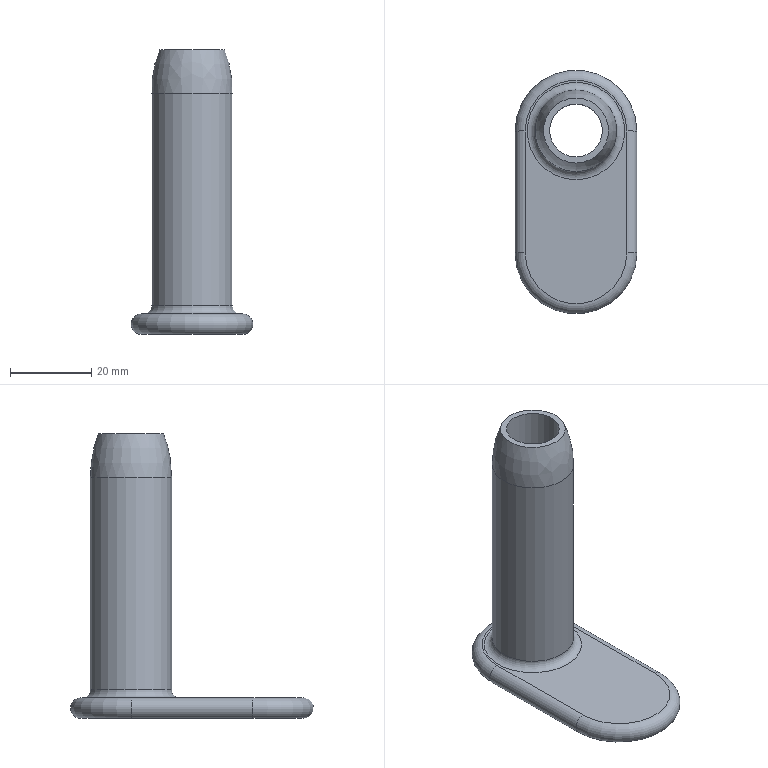Component | NX | UPPER_MOUNT_2 | 1 solid | 14 faces | box 30 x 60 x 70 mm | volume 13408 mm3 | cylinder 5 | plane 3 | torus 3 | cone 2 | spline 1 | commonest cylinder face diameters 5 x2 20 x1 18 x1 13 x1
STEP:
#1=CARTESIAN_POINT('',(0.,0.,0.));
#2=DIRECTION('',(0.,0.,1.));
#3=DIRECTION('',(1.,0.,0.));
#4=AXIS2_PLACEMENT_3D('',#1,#2,#3);
#5=CARTESIAN_POINT('',(-270.,134.875,-190.));
#6=VERTEX_POINT('',#5);
#7=CARTESIAN_POINT('',(-270.,124.875,-190.));
#8=DIRECTION('',(0.,0.,1.));
#9=DIRECTION('',(0.,1.,0.));
#10=AXIS2_PLACEMENT_3D('',#7,#8,#9);
#11=CIRCLE('',#10,10.);
#12=CARTESIAN_POINT('',(-270.,94.875,-190.));
#13=DIRECTION('',(0.,0.,1.));
#14=DIRECTION('',(0.,1.,0.));
#15=AXIS2_PLACEMENT_3D('',#12,#13,#14);
#16=PLANE('',#15);
#17=CARTESIAN_POINT('',(30.,0.));
#18=DIRECTION('',(1.,0.));
#19=AXIS2_PLACEMENT_2D('',#17,#18);
#20=CIRCLE('',#19,10.);
#21=(GEOMETRIC_REPRESENTATION_CONTEXT(2)PARAMETRIC_REPRESENTATION_CONTEXT()REPRESENTATION_CONTEXT('',''));
#22=DEFINITIONAL_REPRESENTATION('',(#20),#21);
#23=PCURVE('',#16,#22);
#24=CARTESIAN_POINT('',(-270.,124.875,-190.));
#25=DIRECTION('',(0.,0.,-1.));
#26=DIRECTION('',(0.,-1.,0.));
#27=AXIS2_PLACEMENT_3D('',#24,#25,#26);
#28=CONICAL_SURFACE('',#27,10.,0.7854);
#29=CARTESIAN_POINT('',(9.425,0.));
#30=DIRECTION('',(-1.,0.));
#31=VECTOR('',#30,1.);
#32=LINE('',#29,#31);
#33=(GEOMETRIC_REPRESENTATION_CONTEXT(2)PARAMETRIC_REPRESENTATION_CONTEXT()REPRESENTATION_CONTEXT('',''));
#34=DEFINITIONAL_REPRESENTATION('',(#32),#33);
#35=PCURVE('',#28,#34);
#36=SURFACE_CURVE('',#11,(#23,#35),.PCURVE_S1.);
#37=EDGE_CURVE('',#6,#6,#36,.T.);
#38=ORIENTED_EDGE('',*,*,#37,.T.);
#39=EDGE_LOOP('',(#38));
#40=FACE_BOUND('',#39,.T.);
#41=CARTESIAN_POINT('',(-282.5,94.875,-190.));
#42=VERTEX_POINT('',#41);
#43=CARTESIAN_POINT('',(-282.5,124.875,-190.));
#44=VERTEX_POINT('',#43);
#45=CARTESIAN_POINT('',(-282.5,124.875,-190.));
#46=DIRECTION('',(0.,1.,0.));
#47=VECTOR('',#46,1.);
#48=LINE('',#45,#47);
#49=CARTESIAN_POINT('',(30.,12.5));
#50=DIRECTION('',(1.,0.));
#51=VECTOR('',#50,1.);
#52=LINE('',#49,#51);
#53=(GEOMETRIC_REPRESENTATION_CONTEXT(2)PARAMETRIC_REPRESENTATION_CONTEXT()REPRESENTATION_CONTEXT('',''));
#54=DEFINITIONAL_REPRESENTATION('',(#52),#53);
#55=PCURVE('',#16,#54);
#56=CARTESIAN_POINT('',(-282.5,124.875,-187.5));
#57=DIRECTION('',(0.,1.,0.));
#58=DIRECTION('',(0.,0.,-1.));
#59=AXIS2_PLACEMENT_3D('',#56,#57,#58);
#60=CYLINDRICAL_SURFACE('',#59,2.5);
#61=CARTESIAN_POINT('',(0.,0.));
#62=DIRECTION('',(0.,1.));
#63=VECTOR('',#62,1.);
#64=LINE('',#61,#63);
#65=(GEOMETRIC_REPRESENTATION_CONTEXT(2)PARAMETRIC_REPRESENTATION_CONTEXT()REPRESENTATION_CONTEXT('',''));
#66=DEFINITIONAL_REPRESENTATION('',(#64),#65);
#67=PCURVE('',#60,#66);
#68=SURFACE_CURVE('',#48,(#55,#67),.PCURVE_S1.);
#69=EDGE_CURVE('',#42,#44,#68,.T.);
#70=ORIENTED_EDGE('',*,*,#69,.T.);
#71=CARTESIAN_POINT('',(-257.5,124.875,-190.));
#72=VERTEX_POINT('',#71);
#73=CARTESIAN_POINT('',(-270.,124.875,-190.));
#74=DIRECTION('',(0.,0.,-1.));
#75=DIRECTION('',(0.,1.,0.));
#76=AXIS2_PLACEMENT_3D('',#73,#74,#75);
#77=CIRCLE('',#76,12.5);
#78=CARTESIAN_POINT('',(42.5,0.));
#79=CARTESIAN_POINT('',(42.5,-21.651));
#80=CARTESIAN_POINT('',(23.75,-10.825));
#81=CARTESIAN_POINT('',(5.,-0.));
#82=CARTESIAN_POINT('',(23.75,10.825));
#83=CARTESIAN_POINT('',(42.5,21.651));
#84=CARTESIAN_POINT('',(42.5,0.));
#85=(BOUNDED_CURVE()B_SPLINE_CURVE(2,(#78,#79,#80,#81,#82,#83,#84),.UNSPECIFIED.,.T.,.F.)B_SPLINE_CURVE_WITH_KNOTS((1,2,2,2,2,1),(-2.094,0.,2.094,4.189,6.283,8.378),.UNSPECIFIED.)CURVE()GEOMETRIC_REPRESENTATION_ITEM()RATIONAL_B_SPLINE_CURVE((1.,0.5,1.,0.5,1.,0.5,1.))REPRESENTATION_ITEM(''));
#86=(GEOMETRIC_REPRESENTATION_CONTEXT(2)PARAMETRIC_REPRESENTATION_CONTEXT()REPRESENTATION_CONTEXT('',''));
#87=DEFINITIONAL_REPRESENTATION('',(#85),#86);
#88=PCURVE('',#16,#87);
#89=CARTESIAN_POINT('',(-270.,124.875,-187.5));
#90=DIRECTION('',(0.,0.,1.));
#91=DIRECTION('',(0.,1.,0.));
#92=AXIS2_PLACEMENT_3D('',#89,#90,#91);
#93=TOROIDAL_SURFACE('',#92,12.5,2.5);
#94=CARTESIAN_POINT('',(12.566,-1.571));
#95=DIRECTION('',(-1.,0.));
#96=VECTOR('',#95,1.);
#97=LINE('',#94,#96);
#98=(GEOMETRIC_REPRESENTATION_CONTEXT(2)PARAMETRIC_REPRESENTATION_CONTEXT()REPRESENTATION_CONTEXT('',''));
#99=DEFINITIONAL_REPRESENTATION('',(#97),#98);
#100=PCURVE('',#93,#99);
#101=SURFACE_CURVE('',#77,(#88,#100),.PCURVE_S1.);
#102=EDGE_CURVE('',#44,#72,#101,.T.);
#103=ORIENTED_EDGE('',*,*,#102,.T.);
#104=CARTESIAN_POINT('',(-257.5,94.875,-190.));
#105=VERTEX_POINT('',#104);
#106=CARTESIAN_POINT('',(-257.5,94.875,-190.));
#107=DIRECTION('',(0.,-1.,0.));
#108=VECTOR('',#107,1.);
#109=LINE('',#106,#108);
#110=CARTESIAN_POINT('',(0.,-12.5));
#111=DIRECTION('',(-1.,0.));
#112=VECTOR('',#111,1.);
#113=LINE('',#110,#112);
#114=(GEOMETRIC_REPRESENTATION_CONTEXT(2)PARAMETRIC_REPRESENTATION_CONTEXT()REPRESENTATION_CONTEXT('',''));
#115=DEFINITIONAL_REPRESENTATION('',(#113),#114);
#116=PCURVE('',#16,#115);
#117=CARTESIAN_POINT('',(-257.5,94.875,-187.5));
#118=DIRECTION('',(0.,-1.,0.));
#119=DIRECTION('',(0.,0.,1.));
#120=AXIS2_PLACEMENT_3D('',#117,#118,#119);
#121=CYLINDRICAL_SURFACE('',#120,2.5);
#122=CARTESIAN_POINT('',(3.142,0.));
#123=DIRECTION('',(0.,1.));
#124=VECTOR('',#123,1.);
#125=LINE('',#122,#124);
#126=(GEOMETRIC_REPRESENTATION_CONTEXT(2)PARAMETRIC_REPRESENTATION_CONTEXT()REPRESENTATION_CONTEXT('',''));
#127=DEFINITIONAL_REPRESENTATION('',(#125),#126);
#128=PCURVE('',#121,#127);
#129=SURFACE_CURVE('',#109,(#116,#128),.PCURVE_S1.);
#130=EDGE_CURVE('',#72,#105,#129,.T.);
#131=ORIENTED_EDGE('',*,*,#130,.T.);
#132=CARTESIAN_POINT('',(-270.,94.875,-190.));
#133=DIRECTION('',(0.,0.,-1.));
#134=DIRECTION('',(0.,1.,0.));
#135=AXIS2_PLACEMENT_3D('',#132,#133,#134);
#136=CIRCLE('',#135,12.5);
#137=CARTESIAN_POINT('',(12.5,0.));
#138=CARTESIAN_POINT('',(12.5,-21.651));
#139=CARTESIAN_POINT('',(-6.25,-10.825));
#140=CARTESIAN_POINT('',(-25.,-0.));
#141=CARTESIAN_POINT('',(-6.25,10.825));
#142=CARTESIAN_POINT('',(12.5,21.651));
#143=CARTESIAN_POINT('',(12.5,0.));
#144=(BOUNDED_CURVE()B_SPLINE_CURVE(2,(#137,#138,#139,#140,#141,#142,#143),.UNSPECIFIED.,.T.,.F.)B_SPLINE_CURVE_WITH_KNOTS((1,2,2,2,2,1),(-2.094,0.,2.094,4.189,6.283,8.378),.UNSPECIFIED.)CURVE()GEOMETRIC_REPRESENTATION_ITEM()RATIONAL_B_SPLINE_CURVE((1.,0.5,1.,0.5,1.,0.5,1.))REPRESENTATION_ITEM(''));
#145=(GEOMETRIC_REPRESENTATION_CONTEXT(2)PARAMETRIC_REPRESENTATION_CONTEXT()REPRESENTATION_CONTEXT('',''));
#146=DEFINITIONAL_REPRESENTATION('',(#144),#145);
#147=PCURVE('',#16,#146);
#148=CARTESIAN_POINT('',(-270.,94.875,-187.5));
#149=DIRECTION('',(0.,0.,1.));
#150=DIRECTION('',(0.,1.,0.));
#151=AXIS2_PLACEMENT_3D('',#148,#149,#150);
#152=TOROIDAL_SURFACE('',#151,12.5,2.5);
#153=CARTESIAN_POINT('',(6.283,-1.571));
#154=DIRECTION('',(-1.,0.));
#155=VECTOR('',#154,1.);
#156=LINE('',#153,#155);
#157=(GEOMETRIC_REPRESENTATION_CONTEXT(2)PARAMETRIC_REPRESENTATION_CONTEXT()REPRESENTATION_CONTEXT('',''));
#158=DEFINITIONAL_REPRESENTATION('',(#156),#157);
#159=PCURVE('',#152,#158);
#160=SURFACE_CURVE('',#136,(#147,#159),.PCURVE_S1.);
#161=EDGE_CURVE('',#105,#42,#160,.T.);
#162=ORIENTED_EDGE('',*,*,#161,.T.);
#163=EDGE_LOOP('',(#70,#103,#131,#162));
#164=FACE_BOUND('',#163,.T.);
#165=ADVANCED_FACE('',(#40,#164),#16,.F.);
#166=CARTESIAN_POINT('',(-270.,136.875,-185.));
#167=VERTEX_POINT('',#166);
#168=CARTESIAN_POINT('',(-270.,124.875,-185.));
#169=DIRECTION('',(0.,0.,-1.));
#170=DIRECTION('',(0.,1.,0.));
#171=AXIS2_PLACEMENT_3D('',#168,#169,#170);
#172=CIRCLE('',#171,12.);
#173=CARTESIAN_POINT('',(-270.,94.875,-185.));
#174=DIRECTION('',(0.,0.,1.));
#175=DIRECTION('',(0.,1.,0.));
#176=AXIS2_PLACEMENT_3D('',#173,#174,#175);
#177=PLANE('',#176);
#178=CARTESIAN_POINT('',(42.,0.));
#179=CARTESIAN_POINT('',(42.,-20.785));
#180=CARTESIAN_POINT('',(24.,-10.392));
#181=CARTESIAN_POINT('',(6.,-0.));
#182=CARTESIAN_POINT('',(24.,10.392));
#183=CARTESIAN_POINT('',(42.,20.785));
#184=CARTESIAN_POINT('',(42.,0.));
#185=(BOUNDED_CURVE()B_SPLINE_CURVE(2,(#178,#179,#180,#181,#182,#183,#184),.UNSPECIFIED.,.T.,.F.)B_SPLINE_CURVE_WITH_KNOTS((1,2,2,2,2,1),(-2.094,0.,2.094,4.189,6.283,8.378),.UNSPECIFIED.)CURVE()GEOMETRIC_REPRESENTATION_ITEM()RATIONAL_B_SPLINE_CURVE((1.,0.5,1.,0.5,1.,0.5,1.))REPRESENTATION_ITEM(''));
#186=(GEOMETRIC_REPRESENTATION_CONTEXT(2)PARAMETRIC_REPRESENTATION_CONTEXT()REPRESENTATION_CONTEXT('',''));
#187=DEFINITIONAL_REPRESENTATION('',(#185),#186);
#188=PCURVE('',#177,#187);
#189=CARTESIAN_POINT('',(-270.,124.875,-183.));
#190=DIRECTION('',(0.,0.,1.));
#191=DIRECTION('',(0.,1.,0.));
#192=AXIS2_PLACEMENT_3D('',#189,#190,#191);
#193=TOROIDAL_SURFACE('',#192,12.,2.);
#194=CARTESIAN_POINT('',(6.283,4.712));
#195=DIRECTION('',(-1.,0.));
#196=VECTOR('',#195,1.);
#197=LINE('',#194,#196);
#198=(GEOMETRIC_REPRESENTATION_CONTEXT(2)PARAMETRIC_REPRESENTATION_CONTEXT()REPRESENTATION_CONTEXT('',''));
#199=DEFINITIONAL_REPRESENTATION('',(#197),#198);
#200=PCURVE('',#193,#199);
#201=SURFACE_CURVE('',#172,(#188,#200),.PCURVE_S1.);
#202=EDGE_CURVE('',#167,#167,#201,.T.);
#203=ORIENTED_EDGE('',*,*,#202,.T.);
#204=EDGE_LOOP('',(#203));
#205=FACE_BOUND('',#204,.T.);
#206=CARTESIAN_POINT('',(-282.5,94.875,-185.));
#207=VERTEX_POINT('',#206);
#208=CARTESIAN_POINT('',(-257.5,94.875,-185.));
#209=VERTEX_POINT('',#208);
#210=CARTESIAN_POINT('',(-270.,94.875,-185.));
#211=DIRECTION('',(0.,0.,1.));
#212=DIRECTION('',(0.,1.,0.));
#213=AXIS2_PLACEMENT_3D('',#210,#211,#212);
#214=CIRCLE('',#213,12.5);
#215=CARTESIAN_POINT('',(0.,0.));
#216=DIRECTION('',(1.,0.));
#217=AXIS2_PLACEMENT_2D('',#215,#216);
#218=CIRCLE('',#217,12.5);
#219=(GEOMETRIC_REPRESENTATION_CONTEXT(2)PARAMETRIC_REPRESENTATION_CONTEXT()REPRESENTATION_CONTEXT('',''));
#220=DEFINITIONAL_REPRESENTATION('',(#218),#219);
#221=PCURVE('',#177,#220);
#222=CARTESIAN_POINT('',(0.,1.571));
#223=DIRECTION('',(1.,0.));
#224=VECTOR('',#223,1.);
#225=LINE('',#222,#224);
#226=(GEOMETRIC_REPRESENTATION_CONTEXT(2)PARAMETRIC_REPRESENTATION_CONTEXT()REPRESENTATION_CONTEXT('',''));
#227=DEFINITIONAL_REPRESENTATION('',(#225),#226);
#228=PCURVE('',#152,#227);
#229=SURFACE_CURVE('',#214,(#221,#228),.PCURVE_S1.);
#230=EDGE_CURVE('',#207,#209,#229,.T.);
#231=ORIENTED_EDGE('',*,*,#230,.T.);
#232=CARTESIAN_POINT('',(-257.5,124.875,-185.));
#233=VERTEX_POINT('',#232);
#234=CARTESIAN_POINT('',(-257.5,94.875,-185.));
#235=DIRECTION('',(0.,1.,0.));
#236=VECTOR('',#235,1.);
#237=LINE('',#234,#236);
#238=CARTESIAN_POINT('',(0.,-12.5));
#239=DIRECTION('',(1.,0.));
#240=VECTOR('',#239,1.);
#241=LINE('',#238,#240);
#242=(GEOMETRIC_REPRESENTATION_CONTEXT(2)PARAMETRIC_REPRESENTATION_CONTEXT()REPRESENTATION_CONTEXT('',''));
#243=DEFINITIONAL_REPRESENTATION('',(#241),#242);
#244=PCURVE('',#177,#243);
#245=CARTESIAN_POINT('',(6.283,0.));
#246=DIRECTION('',(0.,-1.));
#247=VECTOR('',#246,1.);
#248=LINE('',#245,#247);
#249=(GEOMETRIC_REPRESENTATION_CONTEXT(2)PARAMETRIC_REPRESENTATION_CONTEXT()REPRESENTATION_CONTEXT('',''));
#250=DEFINITIONAL_REPRESENTATION('',(#248),#249);
#251=PCURVE('',#121,#250);
#252=SURFACE_CURVE('',#237,(#244,#251),.PCURVE_S1.);
#253=EDGE_CURVE('',#209,#233,#252,.T.);
#254=ORIENTED_EDGE('',*,*,#253,.T.);
#255=CARTESIAN_POINT('',(-282.5,124.875,-185.));
#256=VERTEX_POINT('',#255);
#257=CARTESIAN_POINT('',(-270.,124.875,-185.));
#258=DIRECTION('',(0.,0.,1.));
#259=DIRECTION('',(0.,1.,0.));
#260=AXIS2_PLACEMENT_3D('',#257,#258,#259);
#261=CIRCLE('',#260,12.5);
#262=CARTESIAN_POINT('',(30.,0.));
#263=DIRECTION('',(1.,0.));
#264=AXIS2_PLACEMENT_2D('',#262,#263);
#265=CIRCLE('',#264,12.5);
#266=(GEOMETRIC_REPRESENTATION_CONTEXT(2)PARAMETRIC_REPRESENTATION_CONTEXT()REPRESENTATION_CONTEXT('',''));
#267=DEFINITIONAL_REPRESENTATION('',(#265),#266);
#268=PCURVE('',#177,#267);
#269=CARTESIAN_POINT('',(0.,1.571));
#270=DIRECTION('',(1.,0.));
#271=VECTOR('',#270,1.);
#272=LINE('',#269,#271);
#273=(GEOMETRIC_REPRESENTATION_CONTEXT(2)PARAMETRIC_REPRESENTATION_CONTEXT()REPRESENTATION_CONTEXT('',''));
#274=DEFINITIONAL_REPRESENTATION('',(#272),#273);
#275=PCURVE('',#93,#274);
#276=SURFACE_CURVE('',#261,(#268,#275),.PCURVE_S1.);
#277=EDGE_CURVE('',#233,#256,#276,.T.);
#278=ORIENTED_EDGE('',*,*,#277,.T.);
#279=CARTESIAN_POINT('',(-282.5,94.875,-185.));
#280=DIRECTION('',(0.,-1.,0.));
#281=VECTOR('',#280,1.);
#282=LINE('',#279,#281);
#283=CARTESIAN_POINT('',(0.,12.5));
#284=DIRECTION('',(-1.,0.));
#285=VECTOR('',#284,1.);
#286=LINE('',#283,#285);
#287=(GEOMETRIC_REPRESENTATION_CONTEXT(2)PARAMETRIC_REPRESENTATION_CONTEXT()REPRESENTATION_CONTEXT('',''));
#288=DEFINITIONAL_REPRESENTATION('',(#286),#287);
#289=PCURVE('',#177,#288);
#290=CARTESIAN_POINT('',(3.142,-30.));
#291=DIRECTION('',(0.,-1.));
#292=VECTOR('',#291,1.);
#293=LINE('',#290,#292);
#294=(GEOMETRIC_REPRESENTATION_CONTEXT(2)PARAMETRIC_REPRESENTATION_CONTEXT()REPRESENTATION_CONTEXT('',''));
#295=DEFINITIONAL_REPRESENTATION('',(#293),#294);
#296=PCURVE('',#60,#295);
#297=SURFACE_CURVE('',#282,(#289,#296),.PCURVE_S1.);
#298=EDGE_CURVE('',#256,#207,#297,.T.);
#299=ORIENTED_EDGE('',*,*,#298,.T.);
#300=EDGE_LOOP('',(#231,#254,#278,#299));
#301=FACE_BOUND('',#300,.T.);
#302=ADVANCED_FACE('',(#205,#301),#177,.T.);
#303=CARTESIAN_POINT('',(-257.5,94.875,-187.5));
#304=DIRECTION('',(0.,1.,0.));
#305=DIRECTION('',(0.,0.,-1.));
#306=AXIS2_PLACEMENT_3D('',#303,#304,#305);
#307=CIRCLE('',#306,2.5);
#308=CARTESIAN_POINT('',(4.712,4.712));
#309=DIRECTION('',(0.,-1.));
#310=VECTOR('',#309,1.);
#311=LINE('',#308,#310);
#312=(GEOMETRIC_REPRESENTATION_CONTEXT(2)PARAMETRIC_REPRESENTATION_CONTEXT()REPRESENTATION_CONTEXT('',''));
#313=DEFINITIONAL_REPRESENTATION('',(#311),#312);
#314=PCURVE('',#152,#313);
#315=CARTESIAN_POINT('',(9.425,0.));
#316=DIRECTION('',(-1.,0.));
#317=VECTOR('',#316,1.);
#318=LINE('',#315,#317);
#319=(GEOMETRIC_REPRESENTATION_CONTEXT(2)PARAMETRIC_REPRESENTATION_CONTEXT()REPRESENTATION_CONTEXT('',''));
#320=DEFINITIONAL_REPRESENTATION('',(#318),#319);
#321=PCURVE('',#121,#320);
#322=SURFACE_CURVE('',#307,(#314,#321),.PCURVE_S1.);
#323=EDGE_CURVE('',#209,#105,#322,.T.);
#324=ORIENTED_EDGE('',*,*,#323,.F.);
#325=ORIENTED_EDGE('',*,*,#230,.F.);
#326=CARTESIAN_POINT('',(-282.5,94.875,-187.5));
#327=DIRECTION('',(0.,1.,0.));
#328=DIRECTION('',(0.,0.,-1.));
#329=AXIS2_PLACEMENT_3D('',#326,#327,#328);
#330=CIRCLE('',#329,2.5);
#331=CARTESIAN_POINT('',(1.571,-1.571));
#332=DIRECTION('',(0.,1.));
#333=VECTOR('',#332,1.);
#334=LINE('',#331,#333);
#335=(GEOMETRIC_REPRESENTATION_CONTEXT(2)PARAMETRIC_REPRESENTATION_CONTEXT()REPRESENTATION_CONTEXT('',''));
#336=DEFINITIONAL_REPRESENTATION('',(#334),#335);
#337=PCURVE('',#152,#336);
#338=CARTESIAN_POINT('',(0.,-30.));
#339=DIRECTION('',(1.,0.));
#340=VECTOR('',#339,1.);
#341=LINE('',#338,#340);
#342=(GEOMETRIC_REPRESENTATION_CONTEXT(2)PARAMETRIC_REPRESENTATION_CONTEXT()REPRESENTATION_CONTEXT('',''));
#343=DEFINITIONAL_REPRESENTATION('',(#341),#342);
#344=PCURVE('',#60,#343);
#345=SURFACE_CURVE('',#330,(#337,#344),.PCURVE_S1.);
#346=EDGE_CURVE('',#42,#207,#345,.T.);
#347=ORIENTED_EDGE('',*,*,#346,.F.);
#348=ORIENTED_EDGE('',*,*,#161,.F.);
#349=EDGE_LOOP('',(#324,#325,#347,#348));
#350=FACE_BOUND('',#349,.T.);
#351=ADVANCED_FACE('',(#350),#152,.T.);
#352=ORIENTED_EDGE('',*,*,#346,.T.);
#353=ORIENTED_EDGE('',*,*,#298,.F.);
#354=CARTESIAN_POINT('',(-282.5,124.875,-187.5));
#355=DIRECTION('',(0.,1.,0.));
#356=DIRECTION('',(0.,0.,-1.));
#357=AXIS2_PLACEMENT_3D('',#354,#355,#356);
#358=CIRCLE('',#357,2.5);
#359=CARTESIAN_POINT('',(0.,0.));
#360=DIRECTION('',(1.,0.));
#361=VECTOR('',#360,1.);
#362=LINE('',#359,#361);
#363=(GEOMETRIC_REPRESENTATION_CONTEXT(2)PARAMETRIC_REPRESENTATION_CONTEXT()REPRESENTATION_CONTEXT('',''));
#364=DEFINITIONAL_REPRESENTATION('',(#362),#363);
#365=PCURVE('',#60,#364);
#366=CARTESIAN_POINT('',(7.854,-1.571));
#367=DIRECTION('',(0.,1.));
#368=VECTOR('',#367,1.);
#369=LINE('',#366,#368);
#370=(GEOMETRIC_REPRESENTATION_CONTEXT(2)PARAMETRIC_REPRESENTATION_CONTEXT()REPRESENTATION_CONTEXT('',''));
#371=DEFINITIONAL_REPRESENTATION('',(#369),#370);
#372=PCURVE('',#93,#371);
#373=SURFACE_CURVE('',#358,(#365,#372),.PCURVE_S1.);
#374=EDGE_CURVE('',#44,#256,#373,.T.);
#375=ORIENTED_EDGE('',*,*,#374,.F.);
#376=ORIENTED_EDGE('',*,*,#69,.F.);
#377=EDGE_LOOP('',(#352,#353,#375,#376));
#378=FACE_BOUND('',#377,.T.);
#379=ADVANCED_FACE('',(#378),#60,.T.);
#380=CARTESIAN_POINT('',(-257.5,124.875,-187.5));
#381=DIRECTION('',(0.,1.,0.));
#382=DIRECTION('',(0.,0.,-1.));
#383=AXIS2_PLACEMENT_3D('',#380,#381,#382);
#384=CIRCLE('',#383,2.5);
#385=CARTESIAN_POINT('',(9.425,-30.));
#386=DIRECTION('',(-1.,0.));
#387=VECTOR('',#386,1.);
#388=LINE('',#385,#387);
#389=(GEOMETRIC_REPRESENTATION_CONTEXT(2)PARAMETRIC_REPRESENTATION_CONTEXT()REPRESENTATION_CONTEXT('',''));
#390=DEFINITIONAL_REPRESENTATION('',(#388),#389);
#391=PCURVE('',#121,#390);
#392=CARTESIAN_POINT('',(4.712,4.712));
#393=DIRECTION('',(0.,-1.));
#394=VECTOR('',#393,1.);
#395=LINE('',#392,#394);
#396=(GEOMETRIC_REPRESENTATION_CONTEXT(2)PARAMETRIC_REPRESENTATION_CONTEXT()REPRESENTATION_CONTEXT('',''));
#397=DEFINITIONAL_REPRESENTATION('',(#395),#396);
#398=PCURVE('',#93,#397);
#399=SURFACE_CURVE('',#384,(#391,#398),.PCURVE_S1.);
#400=EDGE_CURVE('',#233,#72,#399,.T.);
#401=ORIENTED_EDGE('',*,*,#400,.F.);
#402=ORIENTED_EDGE('',*,*,#253,.F.);
#403=ORIENTED_EDGE('',*,*,#323,.T.);
#404=ORIENTED_EDGE('',*,*,#130,.F.);
#405=EDGE_LOOP('',(#401,#402,#403,#404));
#406=FACE_BOUND('',#405,.T.);
#407=ADVANCED_FACE('',(#406),#121,.T.);
#408=ORIENTED_EDGE('',*,*,#277,.F.);
#409=ORIENTED_EDGE('',*,*,#400,.T.);
#410=ORIENTED_EDGE('',*,*,#102,.F.);
#411=ORIENTED_EDGE('',*,*,#374,.T.);
#412=EDGE_LOOP('',(#408,#409,#410,#411));
#413=FACE_BOUND('',#412,.T.);
#414=ADVANCED_FACE('',(#413),#93,.T.);
#415=CARTESIAN_POINT('',(-270.,134.875,-183.));
#416=VERTEX_POINT('',#415);
#417=CARTESIAN_POINT('',(-270.,114.875,-183.));
#418=VERTEX_POINT('',#417);
#419=CARTESIAN_POINT('',(-270.,124.875,-183.));
#420=DIRECTION('',(0.,0.,1.));
#421=DIRECTION('',(0.,1.,0.));
#422=AXIS2_PLACEMENT_3D('',#419,#420,#421);
#423=CIRCLE('',#422,10.);
#424=CARTESIAN_POINT('',(-270.,124.875,-120.));
#425=DIRECTION('',(0.,0.,-1.));
#426=DIRECTION('',(0.,-1.,0.));
#427=AXIS2_PLACEMENT_3D('',#424,#425,#426);
#428=CYLINDRICAL_SURFACE('',#427,10.);
#429=CARTESIAN_POINT('',(3.142,63.));
#430=DIRECTION('',(-1.,0.));
#431=VECTOR('',#430,1.);
#432=LINE('',#429,#431);
#433=(GEOMETRIC_REPRESENTATION_CONTEXT(2)PARAMETRIC_REPRESENTATION_CONTEXT()REPRESENTATION_CONTEXT('',''));
#434=DEFINITIONAL_REPRESENTATION('',(#432),#433);
#435=PCURVE('',#428,#434);
#436=CARTESIAN_POINT('',(0.,3.142));
#437=DIRECTION('',(1.,-0.));
#438=VECTOR('',#437,1.);
#439=LINE('',#436,#438);
#440=(GEOMETRIC_REPRESENTATION_CONTEXT(2)PARAMETRIC_REPRESENTATION_CONTEXT()REPRESENTATION_CONTEXT('',''));
#441=DEFINITIONAL_REPRESENTATION('',(#439),#440);
#442=PCURVE('',#193,#441);
#443=SURFACE_CURVE('',#423,(#435,#442),.PCURVE_S1.);
#444=EDGE_CURVE('',#416,#418,#443,.T.);
#445=ORIENTED_EDGE('',*,*,#444,.T.);
#446=CARTESIAN_POINT('',(-270.,114.875,-130.77));
#447=VERTEX_POINT('',#446);
#448=CARTESIAN_POINT('',(-270.,114.875,-130.77));
#449=CARTESIAN_POINT('',(-270.,114.875,-183.));
#450=B_SPLINE_CURVE_WITH_KNOTS('',1,(#448,#449),.UNSPECIFIED.,.F.,.F.,(2,2),(10.77,63.),.PIECEWISE_BEZIER_KNOTS.);
#451=CARTESIAN_POINT('',(0.,0.));
#452=DIRECTION('',(0.,1.));
#453=VECTOR('',#452,1.);
#454=LINE('',#451,#453);
#455=(GEOMETRIC_REPRESENTATION_CONTEXT(2)PARAMETRIC_REPRESENTATION_CONTEXT()REPRESENTATION_CONTEXT('',''));
#456=DEFINITIONAL_REPRESENTATION('',(#454),#455);
#457=PCURVE('',#428,#456);
#458=CARTESIAN_POINT('',(6.283,0.));
#459=DIRECTION('',(0.,1.));
#460=VECTOR('',#459,1.);
#461=LINE('',#458,#460);
#462=(GEOMETRIC_REPRESENTATION_CONTEXT(2)PARAMETRIC_REPRESENTATION_CONTEXT()REPRESENTATION_CONTEXT('',''));
#463=DEFINITIONAL_REPRESENTATION('',(#461),#462);
#464=PCURVE('',#428,#463);
#465=SEAM_CURVE('',#450,(#457,#464),.PCURVE_S1.);
#466=EDGE_CURVE('',#447,#418,#465,.T.);
#467=ORIENTED_EDGE('',*,*,#466,.F.);
#468=CARTESIAN_POINT('',(-270.,124.875,-130.77));
#469=DIRECTION('',(0.,0.,1.));
#470=DIRECTION('',(0.,-1.,0.));
#471=AXIS2_PLACEMENT_3D('',#468,#469,#470);
#472=CIRCLE('',#471,10.);
#473=CARTESIAN_POINT('',(6.283,10.77));
#474=DIRECTION('',(-1.,0.));
#475=VECTOR('',#474,1.);
#476=LINE('',#473,#475);
#477=(GEOMETRIC_REPRESENTATION_CONTEXT(2)PARAMETRIC_REPRESENTATION_CONTEXT()REPRESENTATION_CONTEXT('',''));
#478=DEFINITIONAL_REPRESENTATION('',(#476),#477);
#479=PCURVE('',#428,#478);
#480=CARTESIAN_POINT('',(-270.,114.875,-130.77));
#481=CARTESIAN_POINT('',(-290.,114.875,-130.77));
#482=CARTESIAN_POINT('',(-290.,134.875,-130.77));
#483=CARTESIAN_POINT('',(-270.,134.875,-130.77));
#484=CARTESIAN_POINT('',(-250.,134.875,-130.77));
#485=CARTESIAN_POINT('',(-250.,114.875,-130.77));
#486=CARTESIAN_POINT('',(-270.,114.875,-130.77));
#487=CARTESIAN_POINT('',(-270.,114.875,-127.077));
#488=CARTESIAN_POINT('',(-290.,114.875,-127.077));
#489=CARTESIAN_POINT('',(-290.,134.875,-127.077));
#490=CARTESIAN_POINT('',(-270.,134.875,-127.077));
#491=CARTESIAN_POINT('',(-250.,134.875,-127.077));
#492=CARTESIAN_POINT('',(-250.,114.875,-127.077));
#493=CARTESIAN_POINT('',(-270.,114.875,-127.077));
#494=CARTESIAN_POINT('',(-270.,115.549,-123.447));
#495=CARTESIAN_POINT('',(-288.652,115.549,-123.447));
#496=CARTESIAN_POINT('',(-288.652,134.201,-123.447));
#497=CARTESIAN_POINT('',(-270.,134.201,-123.447));
#498=CARTESIAN_POINT('',(-251.348,134.201,-123.447));
#499=CARTESIAN_POINT('',(-251.348,115.549,-123.447));
#500=CARTESIAN_POINT('',(-270.,115.549,-123.447));
#501=CARTESIAN_POINT('',(-270.,116.875,-120.));
#502=CARTESIAN_POINT('',(-286.,116.875,-120.));
#503=CARTESIAN_POINT('',(-286.,132.875,-120.));
#504=CARTESIAN_POINT('',(-270.,132.875,-120.));
#505=CARTESIAN_POINT('',(-254.,132.875,-120.));
#506=CARTESIAN_POINT('',(-254.,116.875,-120.));
#507=CARTESIAN_POINT('',(-270.,116.875,-120.));
#508=(BOUNDED_SURFACE()B_SPLINE_SURFACE(3,3,((#480,#481,#482,#483,#484,#485,#486),(#487,#488,#489,#490,#491,#492,#493),(#494,#495,#496,#497,#498,#499,#500),(#501,#502,#503,#504,#505,#506,#507)),.UNSPECIFIED.,.F.,.T.,.F.)B_SPLINE_SURFACE_WITH_KNOTS((4,4),(1,3,3,3,1),(0.,1.),(-0.5,0.,0.5,1.,1.5),.UNSPECIFIED.)GEOMETRIC_REPRESENTATION_ITEM()RATIONAL_B_SPLINE_SURFACE(((1.,0.3333,0.3333,1.,0.3333,0.3333,1.),(0.9888,0.3296,0.3296,0.9888,0.3296,0.3296,0.9888),(0.9888,0.3296,0.3296,0.9888,0.3296,0.3296,0.9888),(1.,0.3333,0.3333,1.,0.3333,0.3333,1.)))REPRESENTATION_ITEM('')SURFACE());
#509=CARTESIAN_POINT('',(0.,1.));
#510=CARTESIAN_POINT('',(0.,0.9765));
#511=CARTESIAN_POINT('',(0.,0.9351));
#512=CARTESIAN_POINT('',(0.,0.8854));
#513=CARTESIAN_POINT('',(0.,0.8425));
#514=CARTESIAN_POINT('',(0.,0.804));
#515=CARTESIAN_POINT('',(0.,0.7678));
#516=CARTESIAN_POINT('',(0.,0.7322));
#517=CARTESIAN_POINT('',(0.,0.696));
#518=CARTESIAN_POINT('',(0.,0.6575));
#519=CARTESIAN_POINT('',(0.,0.6144));
#520=CARTESIAN_POINT('',(0.,0.5657));
#521=CARTESIAN_POINT('',(0.,0.5));
#522=CARTESIAN_POINT('',(0.,0.4343));
#523=CARTESIAN_POINT('',(0.,0.3856));
#524=CARTESIAN_POINT('',(0.,0.3425));
#525=CARTESIAN_POINT('',(0.,0.304));
#526=CARTESIAN_POINT('',(0.,0.2678));
#527=CARTESIAN_POINT('',(0.,0.2322));
#528=CARTESIAN_POINT('',(0.,0.196));
#529=CARTESIAN_POINT('',(0.,0.1575));
#530=CARTESIAN_POINT('',(0.,0.1146));
#531=CARTESIAN_POINT('',(0.,0.06491));
#532=CARTESIAN_POINT('',(0.,0.02352));
#533=CARTESIAN_POINT('',(0.,0.));
#534=B_SPLINE_CURVE_WITH_KNOTS('',3,(#509,#510,#511,#512,#513,#514,#515,#516,#517,#518,#519,#520,#521,#522,#523,#524,#525,#526,#527,#528,#529,#530,#531,#532,#533),.UNSPECIFIED.,.F.,.F.,(4,1,1,1,1,1,1,1,1,1,1,1,1,1,1,1,1,1,1,1,1,1,4),(0.,0.2856,0.5712,0.8568,1.142,1.428,1.714,1.999,2.285,2.57,2.856,3.142,3.427,3.713,3.998,4.284,4.57,4.855,5.141,5.426,5.712,5.998,6.283),.QUASI_UNIFORM_KNOTS.);
#535=(GEOMETRIC_REPRESENTATION_CONTEXT(2)PARAMETRIC_REPRESENTATION_CONTEXT()REPRESENTATION_CONTEXT('',''));
#536=DEFINITIONAL_REPRESENTATION('',(#534),#535);
#537=PCURVE('',#508,#536);
#538=SURFACE_CURVE('',#472,(#479,#537),.PCURVE_S1.);
#539=EDGE_CURVE('',#447,#447,#538,.T.);
#540=ORIENTED_EDGE('',*,*,#539,.F.);
#541=ORIENTED_EDGE('',*,*,#466,.T.);
#542=CARTESIAN_POINT('',(-270.,124.875,-183.));
#543=DIRECTION('',(0.,0.,1.));
#544=DIRECTION('',(0.,1.,0.));
#545=AXIS2_PLACEMENT_3D('',#542,#543,#544);
#546=CIRCLE('',#545,10.);
#547=CARTESIAN_POINT('',(9.425,63.));
#548=DIRECTION('',(-1.,0.));
#549=VECTOR('',#548,1.);
#550=LINE('',#547,#549);
#551=(GEOMETRIC_REPRESENTATION_CONTEXT(2)PARAMETRIC_REPRESENTATION_CONTEXT()REPRESENTATION_CONTEXT('',''));
#552=DEFINITIONAL_REPRESENTATION('',(#550),#551);
#553=PCURVE('',#428,#552);
#554=CARTESIAN_POINT('',(0.,3.142));
#555=DIRECTION('',(1.,0.));
#556=VECTOR('',#555,1.);
#557=LINE('',#554,#556);
#558=(GEOMETRIC_REPRESENTATION_CONTEXT(2)PARAMETRIC_REPRESENTATION_CONTEXT()REPRESENTATION_CONTEXT('',''));
#559=DEFINITIONAL_REPRESENTATION('',(#557),#558);
#560=PCURVE('',#193,#559);
#561=SURFACE_CURVE('',#546,(#553,#560),.PCURVE_S1.);
#562=EDGE_CURVE('',#418,#416,#561,.T.);
#563=ORIENTED_EDGE('',*,*,#562,.T.);
#564=EDGE_LOOP('',(#445,#467,#540,#541,#563));
#565=FACE_BOUND('',#564,.T.);
#566=ADVANCED_FACE('',(#565),#428,.T.);
#567=ORIENTED_EDGE('',*,*,#539,.T.);
#568=CARTESIAN_POINT('',(-270.,116.875,-120.));
#569=VERTEX_POINT('',#568);
#570=CARTESIAN_POINT('',(-270.,114.875,-130.77));
#571=CARTESIAN_POINT('',(-270.,114.875,-127.077));
#572=CARTESIAN_POINT('',(-270.,115.549,-123.447));
#573=CARTESIAN_POINT('',(-270.,116.875,-120.));
#574=(BOUNDED_CURVE()B_SPLINE_CURVE(3,(#570,#571,#572,#573),.UNSPECIFIED.,.F.,.F.)B_SPLINE_CURVE_WITH_KNOTS((4,4),(0.,1.),.PIECEWISE_BEZIER_KNOTS.)CURVE()GEOMETRIC_REPRESENTATION_ITEM()RATIONAL_B_SPLINE_CURVE((1.,0.9888,0.9888,1.))REPRESENTATION_ITEM(''));
#575=CARTESIAN_POINT('',(0.,0.));
#576=DIRECTION('',(1.,0.));
#577=VECTOR('',#576,1.);
#578=LINE('',#575,#577);
#579=(GEOMETRIC_REPRESENTATION_CONTEXT(2)PARAMETRIC_REPRESENTATION_CONTEXT()REPRESENTATION_CONTEXT('',''));
#580=DEFINITIONAL_REPRESENTATION('',(#578),#579);
#581=PCURVE('',#508,#580);
#582=CARTESIAN_POINT('',(0.,1.));
#583=DIRECTION('',(1.,0.));
#584=VECTOR('',#583,1.);
#585=LINE('',#582,#584);
#586=(GEOMETRIC_REPRESENTATION_CONTEXT(2)PARAMETRIC_REPRESENTATION_CONTEXT()REPRESENTATION_CONTEXT('',''));
#587=DEFINITIONAL_REPRESENTATION('',(#585),#586);
#588=PCURVE('',#508,#587);
#589=SEAM_CURVE('',#574,(#581,#588),.PCURVE_S1.);
#590=EDGE_CURVE('',#447,#569,#589,.T.);
#591=ORIENTED_EDGE('',*,*,#590,.T.);
#592=CARTESIAN_POINT('',(-270.,124.875,-120.));
#593=DIRECTION('',(0.,0.,1.));
#594=DIRECTION('',(0.,-1.,0.));
#595=AXIS2_PLACEMENT_3D('',#592,#593,#594);
#596=CIRCLE('',#595,8.);
#597=CARTESIAN_POINT('',(1.,1.));
#598=CARTESIAN_POINT('',(1.,0.9765));
#599=CARTESIAN_POINT('',(1.,0.9351));
#600=CARTESIAN_POINT('',(1.,0.8854));
#601=CARTESIAN_POINT('',(1.,0.8425));
#602=CARTESIAN_POINT('',(1.,0.804));
#603=CARTESIAN_POINT('',(1.,0.7678));
#604=CARTESIAN_POINT('',(1.,0.7322));
#605=CARTESIAN_POINT('',(1.,0.696));
#606=CARTESIAN_POINT('',(1.,0.6575));
#607=CARTESIAN_POINT('',(1.,0.6144));
#608=CARTESIAN_POINT('',(1.,0.5657));
#609=CARTESIAN_POINT('',(1.,0.5));
#610=CARTESIAN_POINT('',(1.,0.4343));
#611=CARTESIAN_POINT('',(1.,0.3856));
#612=CARTESIAN_POINT('',(1.,0.3425));
#613=CARTESIAN_POINT('',(1.,0.304));
#614=CARTESIAN_POINT('',(1.,0.2678));
#615=CARTESIAN_POINT('',(1.,0.2322));
#616=CARTESIAN_POINT('',(1.,0.196));
#617=CARTESIAN_POINT('',(1.,0.1575));
#618=CARTESIAN_POINT('',(1.,0.1146));
#619=CARTESIAN_POINT('',(1.,0.06491));
#620=CARTESIAN_POINT('',(1.,0.02352));
#621=CARTESIAN_POINT('',(1.,0.));
#622=B_SPLINE_CURVE_WITH_KNOTS('',3,(#597,#598,#599,#600,#601,#602,#603,#604,#605,#606,#607,#608,#609,#610,#611,#612,#613,#614,#615,#616,#617,#618,#619,#620,#621),.UNSPECIFIED.,.F.,.F.,(4,1,1,1,1,1,1,1,1,1,1,1,1,1,1,1,1,1,1,1,1,1,4),(0.,0.2856,0.5712,0.8568,1.142,1.428,1.714,1.999,2.285,2.57,2.856,3.142,3.427,3.713,3.998,4.284,4.57,4.855,5.141,5.426,5.712,5.998,6.283),.QUASI_UNIFORM_KNOTS.);
#623=(GEOMETRIC_REPRESENTATION_CONTEXT(2)PARAMETRIC_REPRESENTATION_CONTEXT()REPRESENTATION_CONTEXT('',''));
#624=DEFINITIONAL_REPRESENTATION('',(#622),#623);
#625=PCURVE('',#508,#624);
#626=CARTESIAN_POINT('',(-270.,124.875,-120.));
#627=DIRECTION('',(0.,0.,-1.));
#628=DIRECTION('',(0.,-1.,0.));
#629=AXIS2_PLACEMENT_3D('',#626,#627,#628);
#630=PLANE('',#629);
#631=CARTESIAN_POINT('',(8.,0.));
#632=CARTESIAN_POINT('',(8.,-13.856));
#633=CARTESIAN_POINT('',(-4.,-6.928));
#634=CARTESIAN_POINT('',(-16.,-0.));
#635=CARTESIAN_POINT('',(-4.,6.928));
#636=CARTESIAN_POINT('',(8.,13.856));
#637=CARTESIAN_POINT('',(8.,0.));
#638=(BOUNDED_CURVE()B_SPLINE_CURVE(2,(#631,#632,#633,#634,#635,#636,#637),.UNSPECIFIED.,.T.,.F.)B_SPLINE_CURVE_WITH_KNOTS((1,2,2,2,2,1),(-2.094,0.,2.094,4.189,6.283,8.378),.UNSPECIFIED.)CURVE()GEOMETRIC_REPRESENTATION_ITEM()RATIONAL_B_SPLINE_CURVE((1.,0.5,1.,0.5,1.,0.5,1.))REPRESENTATION_ITEM(''));
#639=(GEOMETRIC_REPRESENTATION_CONTEXT(2)PARAMETRIC_REPRESENTATION_CONTEXT()REPRESENTATION_CONTEXT('',''));
#640=DEFINITIONAL_REPRESENTATION('',(#638),#639);
#641=PCURVE('',#630,#640);
#642=SURFACE_CURVE('',#596,(#625,#641),.PCURVE_S1.);
#643=EDGE_CURVE('',#569,#569,#642,.T.);
#644=ORIENTED_EDGE('',*,*,#643,.F.);
#645=ORIENTED_EDGE('',*,*,#590,.F.);
#646=EDGE_LOOP('',(#567,#591,#644,#645));
#647=FACE_BOUND('',#646,.T.);
#648=ADVANCED_FACE('',(#647),#508,.T.);
#649=CARTESIAN_POINT('',(-270.,118.375,-120.));
#650=VERTEX_POINT('',#649);
#651=CARTESIAN_POINT('',(-270.,124.875,-120.));
#652=DIRECTION('',(0.,0.,-1.));
#653=DIRECTION('',(0.,-1.,0.));
#654=AXIS2_PLACEMENT_3D('',#651,#652,#653);
#655=CIRCLE('',#654,6.5);
#656=CARTESIAN_POINT('',(0.,0.));
#657=DIRECTION('',(1.,0.));
#658=AXIS2_PLACEMENT_2D('',#656,#657);
#659=CIRCLE('',#658,6.5);
#660=(GEOMETRIC_REPRESENTATION_CONTEXT(2)PARAMETRIC_REPRESENTATION_CONTEXT()REPRESENTATION_CONTEXT('',''));
#661=DEFINITIONAL_REPRESENTATION('',(#659),#660);
#662=PCURVE('',#630,#661);
#663=CARTESIAN_POINT('',(-270.,124.875,-120.));
#664=DIRECTION('',(0.,0.,-1.));
#665=DIRECTION('',(0.,-1.,0.));
#666=AXIS2_PLACEMENT_3D('',#663,#664,#665);
#667=CYLINDRICAL_SURFACE('',#666,6.5);
#668=CARTESIAN_POINT('',(0.,0.));
#669=DIRECTION('',(1.,0.));
#670=VECTOR('',#669,1.);
#671=LINE('',#668,#670);
#672=(GEOMETRIC_REPRESENTATION_CONTEXT(2)PARAMETRIC_REPRESENTATION_CONTEXT()REPRESENTATION_CONTEXT('',''));
#673=DEFINITIONAL_REPRESENTATION('',(#671),#672);
#674=PCURVE('',#667,#673);
#675=SURFACE_CURVE('',#655,(#662,#674),.PCURVE_S1.);
#676=EDGE_CURVE('',#650,#650,#675,.T.);
#677=ORIENTED_EDGE('',*,*,#676,.T.);
#678=EDGE_LOOP('',(#677));
#679=FACE_BOUND('',#678,.T.);
#680=ORIENTED_EDGE('',*,*,#643,.T.);
#681=EDGE_LOOP('',(#680));
#682=FACE_BOUND('',#681,.T.);
#683=ADVANCED_FACE('',(#679,#682),#630,.F.);
#684=CARTESIAN_POINT('',(-270.,118.375,-148.498));
#685=VERTEX_POINT('',#684);
#686=CARTESIAN_POINT('',(-270.,124.875,-148.498));
#687=DIRECTION('',(0.,0.,1.));
#688=DIRECTION('',(0.,-1.,0.));
#689=AXIS2_PLACEMENT_3D('',#686,#687,#688);
#690=CIRCLE('',#689,6.5);
#691=CARTESIAN_POINT('',(-270.,124.875,-150.));
#692=DIRECTION('',(0.,0.,-1.));
#693=DIRECTION('',(0.,-1.,0.));
#694=AXIS2_PLACEMENT_3D('',#691,#692,#693);
#695=CONICAL_SURFACE('',#694,9.,1.03);
#696=CARTESIAN_POINT('',(6.283,-1.502));
#697=DIRECTION('',(-1.,0.));
#698=VECTOR('',#697,1.);
#699=LINE('',#696,#698);
#700=(GEOMETRIC_REPRESENTATION_CONTEXT(2)PARAMETRIC_REPRESENTATION_CONTEXT()REPRESENTATION_CONTEXT('',''));
#701=DEFINITIONAL_REPRESENTATION('',(#699),#700);
#702=PCURVE('',#695,#701);
#703=CARTESIAN_POINT('',(6.283,28.498));
#704=DIRECTION('',(-1.,0.));
#705=VECTOR('',#704,1.);
#706=LINE('',#703,#705);
#707=(GEOMETRIC_REPRESENTATION_CONTEXT(2)PARAMETRIC_REPRESENTATION_CONTEXT()REPRESENTATION_CONTEXT('',''));
#708=DEFINITIONAL_REPRESENTATION('',(#706),#707);
#709=PCURVE('',#667,#708);
#710=SURFACE_CURVE('',#690,(#702,#709),.PCURVE_S1.);
#711=EDGE_CURVE('',#685,#685,#710,.T.);
#712=ORIENTED_EDGE('',*,*,#711,.F.);
#713=CARTESIAN_POINT('',(-270.,115.875,-150.));
#714=VERTEX_POINT('',#713);
#715=CARTESIAN_POINT('',(-270.,118.375,-148.498));
#716=CARTESIAN_POINT('',(-270.,115.875,-150.));
#717=B_SPLINE_CURVE_WITH_KNOTS('',1,(#715,#716),.UNSPECIFIED.,.F.,.F.,(2,2),(-2.917,0.),.PIECEWISE_BEZIER_KNOTS.);
#718=CARTESIAN_POINT('',(6.283,0.));
#719=DIRECTION('',(0.,1.));
#720=VECTOR('',#719,1.);
#721=LINE('',#718,#720);
#722=(GEOMETRIC_REPRESENTATION_CONTEXT(2)PARAMETRIC_REPRESENTATION_CONTEXT()REPRESENTATION_CONTEXT('',''));
#723=DEFINITIONAL_REPRESENTATION('',(#721),#722);
#724=PCURVE('',#695,#723);
#725=CARTESIAN_POINT('',(0.,0.));
#726=DIRECTION('',(0.,1.));
#727=VECTOR('',#726,1.);
#728=LINE('',#725,#727);
#729=(GEOMETRIC_REPRESENTATION_CONTEXT(2)PARAMETRIC_REPRESENTATION_CONTEXT()REPRESENTATION_CONTEXT('',''));
#730=DEFINITIONAL_REPRESENTATION('',(#728),#729);
#731=PCURVE('',#695,#730);
#732=SEAM_CURVE('',#717,(#724,#731),.PCURVE_S1.);
#733=EDGE_CURVE('',#685,#714,#732,.T.);
#734=ORIENTED_EDGE('',*,*,#733,.T.);
#735=CARTESIAN_POINT('',(-270.,133.875,-150.));
#736=VERTEX_POINT('',#735);
#737=CARTESIAN_POINT('',(-270.,124.875,-150.));
#738=DIRECTION('',(0.,0.,-1.));
#739=DIRECTION('',(0.,1.,0.));
#740=AXIS2_PLACEMENT_3D('',#737,#738,#739);
#741=CIRCLE('',#740,9.);
#742=CARTESIAN_POINT('',(3.142,0.));
#743=DIRECTION('',(1.,0.));
#744=VECTOR('',#743,1.);
#745=LINE('',#742,#744);
#746=(GEOMETRIC_REPRESENTATION_CONTEXT(2)PARAMETRIC_REPRESENTATION_CONTEXT()REPRESENTATION_CONTEXT('',''));
#747=DEFINITIONAL_REPRESENTATION('',(#745),#746);
#748=PCURVE('',#695,#747);
#749=CARTESIAN_POINT('',(-270.,124.875,-190.));
#750=DIRECTION('',(0.,0.,1.));
#751=DIRECTION('',(0.,1.,0.));
#752=AXIS2_PLACEMENT_3D('',#749,#750,#751);
#753=CYLINDRICAL_SURFACE('',#752,9.);
#754=CARTESIAN_POINT('',(6.283,40.));
#755=DIRECTION('',(-1.,0.));
#756=VECTOR('',#755,1.);
#757=LINE('',#754,#756);
#758=(GEOMETRIC_REPRESENTATION_CONTEXT(2)PARAMETRIC_REPRESENTATION_CONTEXT()REPRESENTATION_CONTEXT('',''));
#759=DEFINITIONAL_REPRESENTATION('',(#757),#758);
#760=PCURVE('',#753,#759);
#761=SURFACE_CURVE('',#741,(#748,#760),.PCURVE_S1.);
#762=EDGE_CURVE('',#736,#714,#761,.T.);
#763=ORIENTED_EDGE('',*,*,#762,.F.);
#764=CARTESIAN_POINT('',(-270.,124.875,-150.));
#765=DIRECTION('',(0.,0.,-1.));
#766=DIRECTION('',(0.,1.,0.));
#767=AXIS2_PLACEMENT_3D('',#764,#765,#766);
#768=CIRCLE('',#767,9.);
#769=CARTESIAN_POINT('',(-3.142,0.));
#770=DIRECTION('',(1.,0.));
#771=VECTOR('',#770,1.);
#772=LINE('',#769,#771);
#773=(GEOMETRIC_REPRESENTATION_CONTEXT(2)PARAMETRIC_REPRESENTATION_CONTEXT()REPRESENTATION_CONTEXT('',''));
#774=DEFINITIONAL_REPRESENTATION('',(#772),#773);
#775=PCURVE('',#695,#774);
#776=CARTESIAN_POINT('',(6.283,40.));
#777=DIRECTION('',(-1.,0.));
#778=VECTOR('',#777,1.);
#779=LINE('',#776,#778);
#780=(GEOMETRIC_REPRESENTATION_CONTEXT(2)PARAMETRIC_REPRESENTATION_CONTEXT()REPRESENTATION_CONTEXT('',''));
#781=DEFINITIONAL_REPRESENTATION('',(#779),#780);
#782=PCURVE('',#753,#781);
#783=SURFACE_CURVE('',#768,(#775,#782),.PCURVE_S1.);
#784=EDGE_CURVE('',#714,#736,#783,.T.);
#785=ORIENTED_EDGE('',*,*,#784,.F.);
#786=ORIENTED_EDGE('',*,*,#733,.F.);
#787=EDGE_LOOP('',(#712,#734,#763,#785,#786));
#788=FACE_BOUND('',#787,.F.);
#789=ADVANCED_FACE('',(#788),#695,.F.);
#790=CARTESIAN_POINT('',(-270.,133.875,-189.));
#791=VERTEX_POINT('',#790);
#792=CARTESIAN_POINT('',(-270.,124.875,-189.));
#793=DIRECTION('',(0.,0.,-1.));
#794=DIRECTION('',(0.,1.,0.));
#795=AXIS2_PLACEMENT_3D('',#792,#793,#794);
#796=CIRCLE('',#795,9.);
#797=CARTESIAN_POINT('',(6.283,1.));
#798=DIRECTION('',(-1.,0.));
#799=VECTOR('',#798,1.);
#800=LINE('',#797,#799);
#801=(GEOMETRIC_REPRESENTATION_CONTEXT(2)PARAMETRIC_REPRESENTATION_CONTEXT()REPRESENTATION_CONTEXT('',''));
#802=DEFINITIONAL_REPRESENTATION('',(#800),#801);
#803=PCURVE('',#753,#802);
#804=CARTESIAN_POINT('',(3.142,-1.));
#805=DIRECTION('',(1.,0.));
#806=VECTOR('',#805,1.);
#807=LINE('',#804,#806);
#808=(GEOMETRIC_REPRESENTATION_CONTEXT(2)PARAMETRIC_REPRESENTATION_CONTEXT()REPRESENTATION_CONTEXT('',''));
#809=DEFINITIONAL_REPRESENTATION('',(#807),#808);
#810=PCURVE('',#28,#809);
#811=SURFACE_CURVE('',#796,(#803,#810),.PCURVE_S1.);
#812=EDGE_CURVE('',#791,#791,#811,.T.);
#813=ORIENTED_EDGE('',*,*,#812,.F.);
#814=CARTESIAN_POINT('',(-270.,133.875,-189.));
#815=CARTESIAN_POINT('',(-270.,133.875,-150.));
#816=B_SPLINE_CURVE_WITH_KNOTS('',1,(#814,#815),.UNSPECIFIED.,.F.,.F.,(2,2),(1.,40.),.PIECEWISE_BEZIER_KNOTS.);
#817=CARTESIAN_POINT('',(6.283,0.));
#818=DIRECTION('',(0.,1.));
#819=VECTOR('',#818,1.);
#820=LINE('',#817,#819);
#821=(GEOMETRIC_REPRESENTATION_CONTEXT(2)PARAMETRIC_REPRESENTATION_CONTEXT()REPRESENTATION_CONTEXT('',''));
#822=DEFINITIONAL_REPRESENTATION('',(#820),#821);
#823=PCURVE('',#753,#822);
#824=CARTESIAN_POINT('',(0.,0.));
#825=DIRECTION('',(0.,1.));
#826=VECTOR('',#825,1.);
#827=LINE('',#824,#826);
#828=(GEOMETRIC_REPRESENTATION_CONTEXT(2)PARAMETRIC_REPRESENTATION_CONTEXT()REPRESENTATION_CONTEXT('',''));
#829=DEFINITIONAL_REPRESENTATION('',(#827),#828);
#830=PCURVE('',#753,#829);
#831=SEAM_CURVE('',#816,(#823,#830),.PCURVE_S1.);
#832=EDGE_CURVE('',#791,#736,#831,.T.);
#833=ORIENTED_EDGE('',*,*,#832,.T.);
#834=ORIENTED_EDGE('',*,*,#762,.T.);
#835=ORIENTED_EDGE('',*,*,#784,.T.);
#836=ORIENTED_EDGE('',*,*,#832,.F.);
#837=EDGE_LOOP('',(#813,#833,#834,#835,#836));
#838=FACE_BOUND('',#837,.F.);
#839=ADVANCED_FACE('',(#838),#753,.F.);
#840=ORIENTED_EDGE('',*,*,#676,.T.);
#841=CARTESIAN_POINT('',(-270.,118.375,-120.));
#842=CARTESIAN_POINT('',(-270.,118.375,-148.498));
#843=B_SPLINE_CURVE_WITH_KNOTS('',1,(#841,#842),.UNSPECIFIED.,.F.,.F.,(2,2),(0.,28.498),.PIECEWISE_BEZIER_KNOTS.);
#844=CARTESIAN_POINT('',(6.283,0.));
#845=DIRECTION('',(0.,1.));
#846=VECTOR('',#845,1.);
#847=LINE('',#844,#846);
#848=(GEOMETRIC_REPRESENTATION_CONTEXT(2)PARAMETRIC_REPRESENTATION_CONTEXT()REPRESENTATION_CONTEXT('',''));
#849=DEFINITIONAL_REPRESENTATION('',(#847),#848);
#850=PCURVE('',#667,#849);
#851=CARTESIAN_POINT('',(0.,0.));
#852=DIRECTION('',(0.,1.));
#853=VECTOR('',#852,1.);
#854=LINE('',#851,#853);
#855=(GEOMETRIC_REPRESENTATION_CONTEXT(2)PARAMETRIC_REPRESENTATION_CONTEXT()REPRESENTATION_CONTEXT('',''));
#856=DEFINITIONAL_REPRESENTATION('',(#854),#855);
#857=PCURVE('',#667,#856);
#858=SEAM_CURVE('',#843,(#850,#857),.PCURVE_S1.);
#859=EDGE_CURVE('',#650,#685,#858,.T.);
#860=ORIENTED_EDGE('',*,*,#859,.T.);
#861=ORIENTED_EDGE('',*,*,#711,.T.);
#862=ORIENTED_EDGE('',*,*,#859,.F.);
#863=EDGE_LOOP('',(#840,#860,#861,#862));
#864=FACE_BOUND('',#863,.F.);
#865=ADVANCED_FACE('',(#864),#667,.F.);
#866=ORIENTED_EDGE('',*,*,#202,.T.);
#867=CARTESIAN_POINT('',(-270.,134.875,-183.));
#868=CARTESIAN_POINT('',(-270.,134.875,-183.535));
#869=CARTESIAN_POINT('',(-270.,135.045,-184.055));
#870=CARTESIAN_POINT('',(-270.,135.371,-184.504));
#871=CARTESIAN_POINT('',(-270.,135.82,-184.83));
#872=CARTESIAN_POINT('',(-270.,136.34,-185.));
#873=CARTESIAN_POINT('',(-270.,136.875,-185.));
#874=(BOUNDED_CURVE()B_SPLINE_CURVE(6,(#867,#868,#869,#870,#871,#872,#873),.UNSPECIFIED.,.F.,.F.)B_SPLINE_CURVE_WITH_KNOTS((7,7),(3.142,4.712),.PIECEWISE_BEZIER_KNOTS.)CURVE()GEOMETRIC_REPRESENTATION_ITEM()RATIONAL_B_SPLINE_CURVE((1.031,1.01,0.9979,0.994,0.9979,1.01,1.031))REPRESENTATION_ITEM(''));
#875=CARTESIAN_POINT('',(0.,0.));
#876=DIRECTION('',(0.,1.));
#877=VECTOR('',#876,1.);
#878=LINE('',#875,#877);
#879=(GEOMETRIC_REPRESENTATION_CONTEXT(2)PARAMETRIC_REPRESENTATION_CONTEXT()REPRESENTATION_CONTEXT('',''));
#880=DEFINITIONAL_REPRESENTATION('',(#878),#879);
#881=PCURVE('',#193,#880);
#882=CARTESIAN_POINT('',(6.283,0.));
#883=DIRECTION('',(0.,1.));
#884=VECTOR('',#883,1.);
#885=LINE('',#882,#884);
#886=(GEOMETRIC_REPRESENTATION_CONTEXT(2)PARAMETRIC_REPRESENTATION_CONTEXT()REPRESENTATION_CONTEXT('',''));
#887=DEFINITIONAL_REPRESENTATION('',(#885),#886);
#888=PCURVE('',#193,#887);
#889=SEAM_CURVE('',#874,(#881,#888),.PCURVE_S1.);
#890=EDGE_CURVE('',#416,#167,#889,.T.);
#891=ORIENTED_EDGE('',*,*,#890,.F.);
#892=ORIENTED_EDGE('',*,*,#444,.T.);
#893=ORIENTED_EDGE('',*,*,#562,.T.);
#894=ORIENTED_EDGE('',*,*,#890,.T.);
#895=EDGE_LOOP('',(#866,#891,#892,#893,#894));
#896=FACE_BOUND('',#895,.F.);
#897=ADVANCED_FACE('',(#896),#193,.F.);
#898=ORIENTED_EDGE('',*,*,#812,.T.);
#899=CARTESIAN_POINT('',(-270.,133.875,-189.));
#900=CARTESIAN_POINT('',(-270.,134.875,-190.));
#901=B_SPLINE_CURVE_WITH_KNOTS('',1,(#899,#900),.UNSPECIFIED.,.F.,.F.,(2,2),(-1.414,0.),.PIECEWISE_BEZIER_KNOTS.);
#902=CARTESIAN_POINT('',(9.425,0.));
#903=DIRECTION('',(0.,1.));
#904=VECTOR('',#903,1.);
#905=LINE('',#902,#904);
#906=(GEOMETRIC_REPRESENTATION_CONTEXT(2)PARAMETRIC_REPRESENTATION_CONTEXT()REPRESENTATION_CONTEXT('',''));
#907=DEFINITIONAL_REPRESENTATION('',(#905),#906);
#908=PCURVE('',#28,#907);
#909=CARTESIAN_POINT('',(3.142,0.));
#910=DIRECTION('',(0.,1.));
#911=VECTOR('',#910,1.);
#912=LINE('',#909,#911);
#913=(GEOMETRIC_REPRESENTATION_CONTEXT(2)PARAMETRIC_REPRESENTATION_CONTEXT()REPRESENTATION_CONTEXT('',''));
#914=DEFINITIONAL_REPRESENTATION('',(#912),#913);
#915=PCURVE('',#28,#914);
#916=SEAM_CURVE('',#901,(#908,#915),.PCURVE_S1.);
#917=EDGE_CURVE('',#791,#6,#916,.T.);
#918=ORIENTED_EDGE('',*,*,#917,.T.);
#919=ORIENTED_EDGE('',*,*,#37,.T.);
#920=ORIENTED_EDGE('',*,*,#917,.F.);
#921=EDGE_LOOP('',(#898,#918,#919,#920));
#922=FACE_BOUND('',#921,.F.);
#923=ADVANCED_FACE('',(#922),#28,.F.);
#924=CLOSED_SHELL('',(#165,#302,#351,#379,#407,#414,#566,#648,#683,#789,#839,#865,#897,#923));
#925=MANIFOLD_SOLID_BREP('',#924);
#926=(LENGTH_UNIT()NAMED_UNIT(*)SI_UNIT(.MILLI.,.METRE.));
#927=UNCERTAINTY_MEASURE_WITH_UNIT(LENGTH_MEASURE(0.000005),#926,'','');
#928=(NAMED_UNIT(*)PLANE_ANGLE_UNIT()SI_UNIT($,.RADIAN.));
#929=(NAMED_UNIT(*)SI_UNIT($,.STERADIAN.)SOLID_ANGLE_UNIT());
#930=(GEOMETRIC_REPRESENTATION_CONTEXT(3)GLOBAL_UNCERTAINTY_ASSIGNED_CONTEXT((#927))GLOBAL_UNIT_ASSIGNED_CONTEXT((#926,#928,#929))REPRESENTATION_CONTEXT('',''));
#931=ADVANCED_BREP_SHAPE_REPRESENTATION('',(#4,#925),#930);